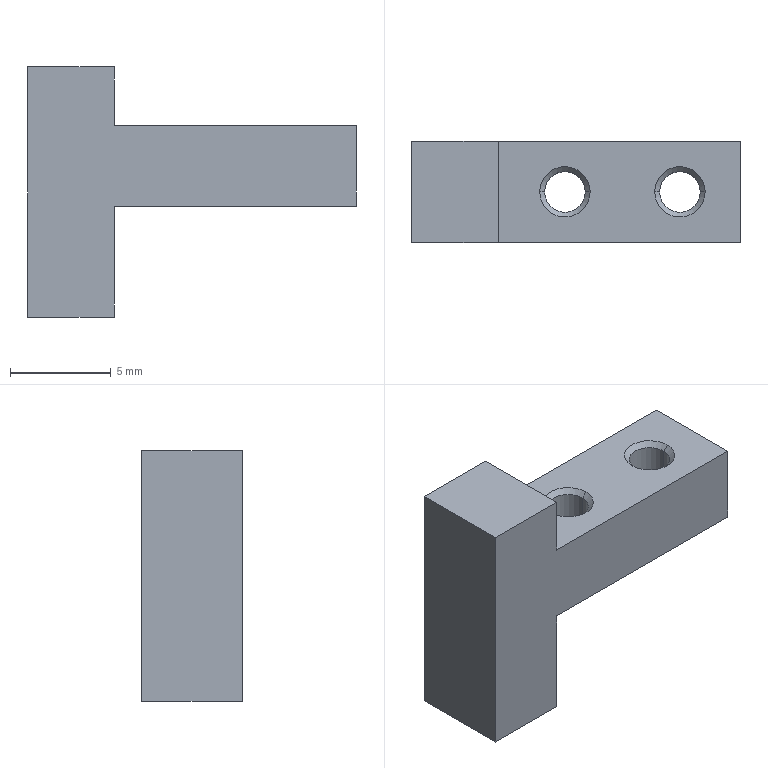Component | SolidWorks | MHZ2-10D-1_CopyCopyFinger2A_MHZ2-10D(11.2)-1 | 1 solid | 22 faces | box 16.3 x 5 x 12.4 mm | volume 480 mm3 | plane 10 | cone 8 | cylinder 4 | commonest cylinder face diameters 2.01 x4
STEP:
#1=COLOUR_RGB('',0.7922,0.8196,0.9333);
#2=FILL_AREA_STYLE_COLOUR('',#1);
#3=FILL_AREA_STYLE('',(#2));
#4=SURFACE_STYLE_FILL_AREA(#3);
#5=SURFACE_SIDE_STYLE('',(#4));
#6=SURFACE_STYLE_USAGE(.BOTH.,#5);
#7=PRESENTATION_STYLE_ASSIGNMENT((#6));
#8=CARTESIAN_POINT('',(7.83,1.719,1.739));
#9=VERTEX_POINT('',#8);
#10=CARTESIAN_POINT('',(7.751,1.719,1.739));
#11=VERTEX_POINT('',#10);
#12=CARTESIAN_POINT('',(7.79,1.719,1.739));
#13=DIRECTION('',(-0.,-0.,-1.));
#14=DIRECTION('',(1.,0.,0.));
#15=AXIS2_PLACEMENT_3D('',#12,#13,#14);
#16=CIRCLE('',#15,0.03957);
#17=EDGE_CURVE('',#9,#11,#16,.T.);
#18=ORIENTED_EDGE('',*,*,#17,.F.);
#19=CARTESIAN_POINT('',(7.839,1.719,1.73));
#20=VERTEX_POINT('',#19);
#21=CARTESIAN_POINT('',(7.839,1.719,1.73));
#22=DIRECTION('',(0.7071,-0.,-0.7071));
#23=VECTOR('',#22,39.37);
#24=LINE('',#21,#23);
#25=EDGE_CURVE('',#9,#20,#24,.T.);
#26=ORIENTED_EDGE('',*,*,#25,.T.);
#27=CARTESIAN_POINT('',(7.741,1.719,1.73));
#28=VERTEX_POINT('',#27);
#29=CARTESIAN_POINT('',(7.79,1.719,1.73));
#30=DIRECTION('',(0.,0.,1.));
#31=DIRECTION('',(-1.,0.,0.));
#32=AXIS2_PLACEMENT_3D('',#29,#30,#31);
#33=CIRCLE('',#32,0.04921);
#34=EDGE_CURVE('',#28,#20,#33,.T.);
#35=ORIENTED_EDGE('',*,*,#34,.F.);
#36=CARTESIAN_POINT('',(7.741,1.719,1.73));
#37=DIRECTION('',(-0.7071,-0.,-0.7071));
#38=VECTOR('',#37,39.37);
#39=LINE('',#36,#38);
#40=EDGE_CURVE('',#11,#28,#39,.T.);
#41=ORIENTED_EDGE('',*,*,#40,.F.);
#42=EDGE_LOOP('',(#18,#26,#35,#41));
#43=FACE_OUTER_BOUND('',#42,.T.);
#44=CARTESIAN_POINT('',(7.79,1.719,1.73));
#45=DIRECTION('',(-0.,-0.,-1.));
#46=DIRECTION('',(-1.,0.,0.));
#47=AXIS2_PLACEMENT_3D('',#44,#45,#46);
#48=CONICAL_SURFACE('',#47,0.04921,0.7854);
#49=ADVANCED_FACE('',(#43),#48,.F.);
#50=CARTESIAN_POINT('',(7.605,1.719,1.739));
#51=VERTEX_POINT('',#50);
#52=CARTESIAN_POINT('',(7.526,1.719,1.739));
#53=VERTEX_POINT('',#52);
#54=CARTESIAN_POINT('',(7.566,1.719,1.739));
#55=DIRECTION('',(-0.,-0.,-1.));
#56=DIRECTION('',(1.,0.,0.));
#57=AXIS2_PLACEMENT_3D('',#54,#55,#56);
#58=CIRCLE('',#57,0.03957);
#59=EDGE_CURVE('',#51,#53,#58,.T.);
#60=ORIENTED_EDGE('',*,*,#59,.F.);
#61=CARTESIAN_POINT('',(7.615,1.719,1.73));
#62=VERTEX_POINT('',#61);
#63=CARTESIAN_POINT('',(7.615,1.719,1.73));
#64=DIRECTION('',(0.7071,-0.,-0.7071));
#65=VECTOR('',#64,39.37);
#66=LINE('',#63,#65);
#67=EDGE_CURVE('',#51,#62,#66,.T.);
#68=ORIENTED_EDGE('',*,*,#67,.T.);
#69=CARTESIAN_POINT('',(7.517,1.719,1.73));
#70=VERTEX_POINT('',#69);
#71=CARTESIAN_POINT('',(7.566,1.719,1.73));
#72=DIRECTION('',(0.,0.,1.));
#73=DIRECTION('',(-1.,0.,0.));
#74=AXIS2_PLACEMENT_3D('',#71,#72,#73);
#75=CIRCLE('',#74,0.04921);
#76=EDGE_CURVE('',#70,#62,#75,.T.);
#77=ORIENTED_EDGE('',*,*,#76,.F.);
#78=CARTESIAN_POINT('',(7.517,1.719,1.73));
#79=DIRECTION('',(-0.7071,-0.,-0.7071));
#80=VECTOR('',#79,39.37);
#81=LINE('',#78,#80);
#82=EDGE_CURVE('',#53,#70,#81,.T.);
#83=ORIENTED_EDGE('',*,*,#82,.F.);
#84=EDGE_LOOP('',(#60,#68,#77,#83));
#85=FACE_OUTER_BOUND('',#84,.T.);
#86=CARTESIAN_POINT('',(7.566,1.719,1.73));
#87=DIRECTION('',(-0.,-0.,-1.));
#88=DIRECTION('',(-1.,0.,0.));
#89=AXIS2_PLACEMENT_3D('',#86,#87,#88);
#90=CONICAL_SURFACE('',#89,0.04921,0.7854);
#91=ADVANCED_FACE('',(#85),#90,.F.);
#92=CARTESIAN_POINT('',(7.751,1.719,1.877));
#93=VERTEX_POINT('',#92);
#94=CARTESIAN_POINT('',(7.83,1.719,1.877));
#95=VERTEX_POINT('',#94);
#96=CARTESIAN_POINT('',(7.79,1.719,1.877));
#97=DIRECTION('',(0.,0.,1.));
#98=DIRECTION('',(1.,0.,0.));
#99=AXIS2_PLACEMENT_3D('',#96,#97,#98);
#100=CIRCLE('',#99,0.03957);
#101=EDGE_CURVE('',#93,#95,#100,.T.);
#102=ORIENTED_EDGE('',*,*,#101,.F.);
#103=CARTESIAN_POINT('',(7.741,1.719,1.887));
#104=VERTEX_POINT('',#103);
#105=CARTESIAN_POINT('',(7.741,1.719,1.887));
#106=DIRECTION('',(-0.7071,0.,0.7071));
#107=VECTOR('',#106,39.37);
#108=LINE('',#105,#107);
#109=EDGE_CURVE('',#93,#104,#108,.T.);
#110=ORIENTED_EDGE('',*,*,#109,.T.);
#111=CARTESIAN_POINT('',(7.839,1.719,1.887));
#112=VERTEX_POINT('',#111);
#113=CARTESIAN_POINT('',(7.79,1.719,1.887));
#114=DIRECTION('',(-0.,-0.,-1.));
#115=DIRECTION('',(1.,0.,0.));
#116=AXIS2_PLACEMENT_3D('',#113,#114,#115);
#117=CIRCLE('',#116,0.04921);
#118=EDGE_CURVE('',#112,#104,#117,.T.);
#119=ORIENTED_EDGE('',*,*,#118,.F.);
#120=CARTESIAN_POINT('',(7.839,1.719,1.887));
#121=DIRECTION('',(0.7071,0.,0.7071));
#122=VECTOR('',#121,39.37);
#123=LINE('',#120,#122);
#124=EDGE_CURVE('',#95,#112,#123,.T.);
#125=ORIENTED_EDGE('',*,*,#124,.F.);
#126=EDGE_LOOP('',(#102,#110,#119,#125));
#127=FACE_OUTER_BOUND('',#126,.T.);
#128=CARTESIAN_POINT('',(7.79,1.719,1.887));
#129=DIRECTION('',(0.,0.,1.));
#130=DIRECTION('',(1.,0.,0.));
#131=AXIS2_PLACEMENT_3D('',#128,#129,#130);
#132=CONICAL_SURFACE('',#131,0.04921,0.7854);
#133=ADVANCED_FACE('',(#127),#132,.F.);
#134=CARTESIAN_POINT('',(7.526,1.719,1.877));
#135=VERTEX_POINT('',#134);
#136=CARTESIAN_POINT('',(7.605,1.719,1.877));
#137=VERTEX_POINT('',#136);
#138=CARTESIAN_POINT('',(7.566,1.719,1.877));
#139=DIRECTION('',(0.,0.,1.));
#140=DIRECTION('',(1.,0.,0.));
#141=AXIS2_PLACEMENT_3D('',#138,#139,#140);
#142=CIRCLE('',#141,0.03957);
#143=EDGE_CURVE('',#135,#137,#142,.T.);
#144=ORIENTED_EDGE('',*,*,#143,.F.);
#145=CARTESIAN_POINT('',(7.517,1.719,1.887));
#146=VERTEX_POINT('',#145);
#147=CARTESIAN_POINT('',(7.517,1.719,1.887));
#148=DIRECTION('',(-0.7071,0.,0.7071));
#149=VECTOR('',#148,39.37);
#150=LINE('',#147,#149);
#151=EDGE_CURVE('',#135,#146,#150,.T.);
#152=ORIENTED_EDGE('',*,*,#151,.T.);
#153=CARTESIAN_POINT('',(7.615,1.719,1.887));
#154=VERTEX_POINT('',#153);
#155=CARTESIAN_POINT('',(7.566,1.719,1.887));
#156=DIRECTION('',(-0.,-0.,-1.));
#157=DIRECTION('',(1.,0.,0.));
#158=AXIS2_PLACEMENT_3D('',#155,#156,#157);
#159=CIRCLE('',#158,0.04921);
#160=EDGE_CURVE('',#154,#146,#159,.T.);
#161=ORIENTED_EDGE('',*,*,#160,.F.);
#162=CARTESIAN_POINT('',(7.615,1.719,1.887));
#163=DIRECTION('',(0.7071,0.,0.7071));
#164=VECTOR('',#163,39.37);
#165=LINE('',#162,#164);
#166=EDGE_CURVE('',#137,#154,#165,.T.);
#167=ORIENTED_EDGE('',*,*,#166,.F.);
#168=EDGE_LOOP('',(#144,#152,#161,#167));
#169=FACE_OUTER_BOUND('',#168,.T.);
#170=CARTESIAN_POINT('',(7.566,1.719,1.887));
#171=DIRECTION('',(0.,0.,1.));
#172=DIRECTION('',(1.,0.,0.));
#173=AXIS2_PLACEMENT_3D('',#170,#171,#172);
#174=CONICAL_SURFACE('',#173,0.04921,0.7854);
#175=ADVANCED_FACE('',(#169),#174,.F.);
#176=ORIENTED_EDGE('',*,*,#101,.T.);
#177=CARTESIAN_POINT('',(7.83,1.719,1.808));
#178=DIRECTION('',(-0.,-0.,-1.));
#179=VECTOR('',#178,39.37);
#180=LINE('',#177,#179);
#181=EDGE_CURVE('',#95,#9,#180,.T.);
#182=ORIENTED_EDGE('',*,*,#181,.T.);
#183=ORIENTED_EDGE('',*,*,#17,.T.);
#184=CARTESIAN_POINT('',(7.751,1.719,1.808));
#185=DIRECTION('',(-0.,-0.,-1.));
#186=VECTOR('',#185,39.37);
#187=LINE('',#184,#186);
#188=EDGE_CURVE('',#93,#11,#187,.T.);
#189=ORIENTED_EDGE('',*,*,#188,.F.);
#190=EDGE_LOOP('',(#176,#182,#183,#189));
#191=FACE_OUTER_BOUND('',#190,.T.);
#192=CARTESIAN_POINT('',(7.79,1.719,1.808));
#193=DIRECTION('',(-0.,-0.,-1.));
#194=DIRECTION('',(-1.,0.,0.));
#195=AXIS2_PLACEMENT_3D('',#192,#193,#194);
#196=CYLINDRICAL_SURFACE('',#195,0.03957);
#197=ADVANCED_FACE('',(#191),#196,.F.);
#198=ORIENTED_EDGE('',*,*,#143,.T.);
#199=CARTESIAN_POINT('',(7.605,1.719,1.808));
#200=DIRECTION('',(-0.,-0.,-1.));
#201=VECTOR('',#200,39.37);
#202=LINE('',#199,#201);
#203=EDGE_CURVE('',#137,#51,#202,.T.);
#204=ORIENTED_EDGE('',*,*,#203,.T.);
#205=ORIENTED_EDGE('',*,*,#59,.T.);
#206=CARTESIAN_POINT('',(7.526,1.719,1.808));
#207=DIRECTION('',(-0.,-0.,-1.));
#208=VECTOR('',#207,39.37);
#209=LINE('',#206,#208);
#210=EDGE_CURVE('',#135,#53,#209,.T.);
#211=ORIENTED_EDGE('',*,*,#210,.F.);
#212=EDGE_LOOP('',(#198,#204,#205,#211));
#213=FACE_OUTER_BOUND('',#212,.T.);
#214=CARTESIAN_POINT('',(7.566,1.719,1.808));
#215=DIRECTION('',(-0.,-0.,-1.));
#216=DIRECTION('',(-1.,0.,0.));
#217=AXIS2_PLACEMENT_3D('',#214,#215,#216);
#218=CYLINDRICAL_SURFACE('',#217,0.03957);
#219=ADVANCED_FACE('',(#213),#218,.F.);
#220=CARTESIAN_POINT('',(7.267,1.818,1.513));
#221=VERTEX_POINT('',#220);
#222=CARTESIAN_POINT('',(7.267,1.818,2.001));
#223=VERTEX_POINT('',#222);
#224=CARTESIAN_POINT('',(7.267,1.818,1.509));
#225=DIRECTION('',(0.,0.,1.));
#226=VECTOR('',#225,39.37);
#227=LINE('',#224,#226);
#228=EDGE_CURVE('',#221,#223,#227,.T.);
#229=ORIENTED_EDGE('',*,*,#228,.T.);
#230=CARTESIAN_POINT('',(7.436,1.818,2.001));
#231=VERTEX_POINT('',#230);
#232=CARTESIAN_POINT('',(7.389,1.818,2.001));
#233=DIRECTION('',(1.,0.,-0.));
#234=VECTOR('',#233,39.37);
#235=LINE('',#232,#234);
#236=EDGE_CURVE('',#223,#231,#235,.T.);
#237=ORIENTED_EDGE('',*,*,#236,.T.);
#238=CARTESIAN_POINT('',(7.436,1.818,1.887));
#239=VERTEX_POINT('',#238);
#240=CARTESIAN_POINT('',(7.436,1.818,1.509));
#241=DIRECTION('',(-0.,-0.,-1.));
#242=VECTOR('',#241,39.37);
#243=LINE('',#240,#242);
#244=EDGE_CURVE('',#231,#239,#243,.T.);
#245=ORIENTED_EDGE('',*,*,#244,.T.);
#246=CARTESIAN_POINT('',(7.908,1.818,1.887));
#247=VERTEX_POINT('',#246);
#248=CARTESIAN_POINT('',(7.389,1.818,1.887));
#249=DIRECTION('',(1.,0.,-0.));
#250=VECTOR('',#249,39.37);
#251=LINE('',#248,#250);
#252=EDGE_CURVE('',#239,#247,#251,.T.);
#253=ORIENTED_EDGE('',*,*,#252,.T.);
#254=CARTESIAN_POINT('',(7.908,1.818,1.73));
#255=VERTEX_POINT('',#254);
#256=CARTESIAN_POINT('',(7.908,1.818,1.509));
#257=DIRECTION('',(-0.,-0.,-1.));
#258=VECTOR('',#257,39.37);
#259=LINE('',#256,#258);
#260=EDGE_CURVE('',#247,#255,#259,.T.);
#261=ORIENTED_EDGE('',*,*,#260,.T.);
#262=CARTESIAN_POINT('',(7.436,1.818,1.73));
#263=VERTEX_POINT('',#262);
#264=CARTESIAN_POINT('',(7.389,1.818,1.73));
#265=DIRECTION('',(-1.,-0.,0.));
#266=VECTOR('',#265,39.37);
#267=LINE('',#264,#266);
#268=EDGE_CURVE('',#255,#263,#267,.T.);
#269=ORIENTED_EDGE('',*,*,#268,.T.);
#270=CARTESIAN_POINT('',(7.436,1.818,1.513));
#271=VERTEX_POINT('',#270);
#272=CARTESIAN_POINT('',(7.436,1.818,1.509));
#273=DIRECTION('',(-0.,-0.,-1.));
#274=VECTOR('',#273,39.37);
#275=LINE('',#272,#274);
#276=EDGE_CURVE('',#263,#271,#275,.T.);
#277=ORIENTED_EDGE('',*,*,#276,.T.);
#278=CARTESIAN_POINT('',(7.389,1.818,1.513));
#279=DIRECTION('',(-1.,-0.,0.));
#280=VECTOR('',#279,39.37);
#281=LINE('',#278,#280);
#282=EDGE_CURVE('',#271,#221,#281,.T.);
#283=ORIENTED_EDGE('',*,*,#282,.T.);
#284=EDGE_LOOP('',(#229,#237,#245,#253,#261,#269,#277,#283));
#285=FACE_OUTER_BOUND('',#284,.T.);
#286=CARTESIAN_POINT('',(7.389,1.818,1.509));
#287=DIRECTION('',(-0.,1.,-0.));
#288=DIRECTION('',(1.,0.,-0.));
#289=AXIS2_PLACEMENT_3D('',#286,#287,#288);
#290=PLANE('',#289);
#291=ADVANCED_FACE('',(#285),#290,.T.);
#292=ORIENTED_EDGE('',*,*,#236,.F.);
#293=CARTESIAN_POINT('',(7.267,1.621,2.001));
#294=VERTEX_POINT('',#293);
#295=CARTESIAN_POINT('',(7.267,1.818,2.001));
#296=DIRECTION('',(0.,-1.,0.));
#297=VECTOR('',#296,39.37);
#298=LINE('',#295,#297);
#299=EDGE_CURVE('',#223,#294,#298,.T.);
#300=ORIENTED_EDGE('',*,*,#299,.T.);
#301=CARTESIAN_POINT('',(7.436,1.621,2.001));
#302=VERTEX_POINT('',#301);
#303=CARTESIAN_POINT('',(7.267,1.621,2.001));
#304=DIRECTION('',(1.,0.,-0.));
#305=VECTOR('',#304,39.37);
#306=LINE('',#303,#305);
#307=EDGE_CURVE('',#294,#302,#306,.T.);
#308=ORIENTED_EDGE('',*,*,#307,.T.);
#309=CARTESIAN_POINT('',(7.436,1.818,2.001));
#310=DIRECTION('',(-0.,1.,-0.));
#311=VECTOR('',#310,39.37);
#312=LINE('',#309,#311);
#313=EDGE_CURVE('',#302,#231,#312,.T.);
#314=ORIENTED_EDGE('',*,*,#313,.T.);
#315=EDGE_LOOP('',(#292,#300,#308,#314));
#316=FACE_OUTER_BOUND('',#315,.T.);
#317=CARTESIAN_POINT('',(7.267,1.818,2.001));
#318=DIRECTION('',(0.,0.,1.));
#319=DIRECTION('',(1.,0.,-0.));
#320=AXIS2_PLACEMENT_3D('',#317,#318,#319);
#321=PLANE('',#320);
#322=ADVANCED_FACE('',(#316),#321,.T.);
#323=ORIENTED_EDGE('',*,*,#228,.F.);
#324=CARTESIAN_POINT('',(7.267,1.621,1.513));
#325=VERTEX_POINT('',#324);
#326=CARTESIAN_POINT('',(7.267,1.818,1.513));
#327=DIRECTION('',(0.,-1.,0.));
#328=VECTOR('',#327,39.37);
#329=LINE('',#326,#328);
#330=EDGE_CURVE('',#221,#325,#329,.T.);
#331=ORIENTED_EDGE('',*,*,#330,.T.);
#332=CARTESIAN_POINT('',(7.267,1.621,1.513));
#333=DIRECTION('',(-0.,0.,1.));
#334=VECTOR('',#333,39.37);
#335=LINE('',#332,#334);
#336=EDGE_CURVE('',#325,#294,#335,.T.);
#337=ORIENTED_EDGE('',*,*,#336,.T.);
#338=ORIENTED_EDGE('',*,*,#299,.F.);
#339=EDGE_LOOP('',(#323,#331,#337,#338));
#340=FACE_OUTER_BOUND('',#339,.T.);
#341=CARTESIAN_POINT('',(7.267,1.818,1.513));
#342=DIRECTION('',(-1.,-0.,-0.));
#343=DIRECTION('',(-0.,0.,1.));
#344=AXIS2_PLACEMENT_3D('',#341,#342,#343);
#345=PLANE('',#344);
#346=ADVANCED_FACE('',(#340),#345,.T.);
#347=ORIENTED_EDGE('',*,*,#282,.F.);
#348=CARTESIAN_POINT('',(7.436,1.621,1.513));
#349=VERTEX_POINT('',#348);
#350=CARTESIAN_POINT('',(7.436,1.818,1.513));
#351=DIRECTION('',(0.,-1.,0.));
#352=VECTOR('',#351,39.37);
#353=LINE('',#350,#352);
#354=EDGE_CURVE('',#271,#349,#353,.T.);
#355=ORIENTED_EDGE('',*,*,#354,.T.);
#356=CARTESIAN_POINT('',(7.436,1.621,1.513));
#357=DIRECTION('',(-1.,-0.,0.));
#358=VECTOR('',#357,39.37);
#359=LINE('',#356,#358);
#360=EDGE_CURVE('',#349,#325,#359,.T.);
#361=ORIENTED_EDGE('',*,*,#360,.T.);
#362=ORIENTED_EDGE('',*,*,#330,.F.);
#363=EDGE_LOOP('',(#347,#355,#361,#362));
#364=FACE_OUTER_BOUND('',#363,.T.);
#365=CARTESIAN_POINT('',(7.436,1.818,1.513));
#366=DIRECTION('',(-0.,-0.,-1.));
#367=DIRECTION('',(-1.,-0.,0.));
#368=AXIS2_PLACEMENT_3D('',#365,#366,#367);
#369=PLANE('',#368);
#370=ADVANCED_FACE('',(#364),#369,.T.);
#371=ORIENTED_EDGE('',*,*,#276,.F.);
#372=CARTESIAN_POINT('',(7.436,1.621,1.73));
#373=VERTEX_POINT('',#372);
#374=CARTESIAN_POINT('',(7.436,1.818,1.73));
#375=DIRECTION('',(0.,-1.,0.));
#376=VECTOR('',#375,39.37);
#377=LINE('',#374,#376);
#378=EDGE_CURVE('',#263,#373,#377,.T.);
#379=ORIENTED_EDGE('',*,*,#378,.T.);
#380=CARTESIAN_POINT('',(7.436,1.621,1.73));
#381=DIRECTION('',(-0.,-0.,-1.));
#382=VECTOR('',#381,39.37);
#383=LINE('',#380,#382);
#384=EDGE_CURVE('',#373,#349,#383,.T.);
#385=ORIENTED_EDGE('',*,*,#384,.T.);
#386=ORIENTED_EDGE('',*,*,#354,.F.);
#387=EDGE_LOOP('',(#371,#379,#385,#386));
#388=FACE_OUTER_BOUND('',#387,.T.);
#389=CARTESIAN_POINT('',(7.436,1.818,1.73));
#390=DIRECTION('',(1.,0.,-0.));
#391=DIRECTION('',(0.,-1.,0.));
#392=AXIS2_PLACEMENT_3D('',#389,#390,#391);
#393=PLANE('',#392);
#394=ADVANCED_FACE('',(#388),#393,.T.);
#395=ORIENTED_EDGE('',*,*,#268,.F.);
#396=CARTESIAN_POINT('',(7.908,1.621,1.73));
#397=VERTEX_POINT('',#396);
#398=CARTESIAN_POINT('',(7.908,1.818,1.73));
#399=DIRECTION('',(0.,-1.,0.));
#400=VECTOR('',#399,39.37);
#401=LINE('',#398,#400);
#402=EDGE_CURVE('',#255,#397,#401,.T.);
#403=ORIENTED_EDGE('',*,*,#402,.T.);
#404=CARTESIAN_POINT('',(7.908,1.621,1.73));
#405=DIRECTION('',(-1.,-0.,0.));
#406=VECTOR('',#405,39.37);
#407=LINE('',#404,#406);
#408=EDGE_CURVE('',#397,#373,#407,.T.);
#409=ORIENTED_EDGE('',*,*,#408,.T.);
#410=ORIENTED_EDGE('',*,*,#378,.F.);
#411=EDGE_LOOP('',(#395,#403,#409,#410));
#412=FACE_OUTER_BOUND('',#411,.T.);
#413=ORIENTED_EDGE('',*,*,#34,.T.);
#414=CARTESIAN_POINT('',(7.79,1.719,1.73));
#415=DIRECTION('',(0.,0.,1.));
#416=DIRECTION('',(-1.,0.,0.));
#417=AXIS2_PLACEMENT_3D('',#414,#415,#416);
#418=CIRCLE('',#417,0.04921);
#419=EDGE_CURVE('',#20,#28,#418,.T.);
#420=ORIENTED_EDGE('',*,*,#419,.T.);
#421=EDGE_LOOP('',(#413,#420));
#422=FACE_BOUND('',#421,.T.);
#423=ORIENTED_EDGE('',*,*,#76,.T.);
#424=CARTESIAN_POINT('',(7.566,1.719,1.73));
#425=DIRECTION('',(0.,0.,1.));
#426=DIRECTION('',(-1.,0.,0.));
#427=AXIS2_PLACEMENT_3D('',#424,#425,#426);
#428=CIRCLE('',#427,0.04921);
#429=EDGE_CURVE('',#62,#70,#428,.T.);
#430=ORIENTED_EDGE('',*,*,#429,.T.);
#431=EDGE_LOOP('',(#423,#430));
#432=FACE_BOUND('',#431,.T.);
#433=CARTESIAN_POINT('',(7.908,1.818,1.73));
#434=DIRECTION('',(-0.,-0.,-1.));
#435=DIRECTION('',(-1.,-0.,0.));
#436=AXIS2_PLACEMENT_3D('',#433,#434,#435);
#437=PLANE('',#436);
#438=ADVANCED_FACE('',(#412,#422,#432),#437,.T.);
#439=ORIENTED_EDGE('',*,*,#260,.F.);
#440=CARTESIAN_POINT('',(7.908,1.621,1.887));
#441=VERTEX_POINT('',#440);
#442=CARTESIAN_POINT('',(7.908,1.818,1.887));
#443=DIRECTION('',(0.,-1.,0.));
#444=VECTOR('',#443,39.37);
#445=LINE('',#442,#444);
#446=EDGE_CURVE('',#247,#441,#445,.T.);
#447=ORIENTED_EDGE('',*,*,#446,.T.);
#448=CARTESIAN_POINT('',(7.908,1.621,1.887));
#449=DIRECTION('',(-0.,-0.,-1.));
#450=VECTOR('',#449,39.37);
#451=LINE('',#448,#450);
#452=EDGE_CURVE('',#441,#397,#451,.T.);
#453=ORIENTED_EDGE('',*,*,#452,.T.);
#454=ORIENTED_EDGE('',*,*,#402,.F.);
#455=EDGE_LOOP('',(#439,#447,#453,#454));
#456=FACE_OUTER_BOUND('',#455,.T.);
#457=CARTESIAN_POINT('',(7.908,1.818,1.887));
#458=DIRECTION('',(1.,0.,-0.));
#459=DIRECTION('',(-0.,-0.,-1.));
#460=AXIS2_PLACEMENT_3D('',#457,#458,#459);
#461=PLANE('',#460);
#462=ADVANCED_FACE('',(#456),#461,.T.);
#463=ORIENTED_EDGE('',*,*,#252,.F.);
#464=CARTESIAN_POINT('',(7.436,1.621,1.887));
#465=VERTEX_POINT('',#464);
#466=CARTESIAN_POINT('',(7.436,1.818,1.887));
#467=DIRECTION('',(0.,-1.,0.));
#468=VECTOR('',#467,39.37);
#469=LINE('',#466,#468);
#470=EDGE_CURVE('',#239,#465,#469,.T.);
#471=ORIENTED_EDGE('',*,*,#470,.T.);
#472=CARTESIAN_POINT('',(7.436,1.621,1.887));
#473=DIRECTION('',(1.,0.,-0.));
#474=VECTOR('',#473,39.37);
#475=LINE('',#472,#474);
#476=EDGE_CURVE('',#465,#441,#475,.T.);
#477=ORIENTED_EDGE('',*,*,#476,.T.);
#478=ORIENTED_EDGE('',*,*,#446,.F.);
#479=EDGE_LOOP('',(#463,#471,#477,#478));
#480=FACE_OUTER_BOUND('',#479,.T.);
#481=ORIENTED_EDGE('',*,*,#118,.T.);
#482=CARTESIAN_POINT('',(7.79,1.719,1.887));
#483=DIRECTION('',(-0.,-0.,-1.));
#484=DIRECTION('',(1.,0.,0.));
#485=AXIS2_PLACEMENT_3D('',#482,#483,#484);
#486=CIRCLE('',#485,0.04921);
#487=EDGE_CURVE('',#104,#112,#486,.T.);
#488=ORIENTED_EDGE('',*,*,#487,.T.);
#489=EDGE_LOOP('',(#481,#488));
#490=FACE_BOUND('',#489,.T.);
#491=ORIENTED_EDGE('',*,*,#160,.T.);
#492=CARTESIAN_POINT('',(7.566,1.719,1.887));
#493=DIRECTION('',(-0.,-0.,-1.));
#494=DIRECTION('',(1.,0.,0.));
#495=AXIS2_PLACEMENT_3D('',#492,#493,#494);
#496=CIRCLE('',#495,0.04921);
#497=EDGE_CURVE('',#146,#154,#496,.T.);
#498=ORIENTED_EDGE('',*,*,#497,.T.);
#499=EDGE_LOOP('',(#491,#498));
#500=FACE_BOUND('',#499,.T.);
#501=CARTESIAN_POINT('',(7.436,1.818,1.887));
#502=DIRECTION('',(0.,0.,1.));
#503=DIRECTION('',(1.,0.,-0.));
#504=AXIS2_PLACEMENT_3D('',#501,#502,#503);
#505=PLANE('',#504);
#506=ADVANCED_FACE('',(#480,#490,#500),#505,.T.);
#507=ORIENTED_EDGE('',*,*,#244,.F.);
#508=ORIENTED_EDGE('',*,*,#313,.F.);
#509=CARTESIAN_POINT('',(7.436,1.621,2.001));
#510=DIRECTION('',(-0.,-0.,-1.));
#511=VECTOR('',#510,39.37);
#512=LINE('',#509,#511);
#513=EDGE_CURVE('',#302,#465,#512,.T.);
#514=ORIENTED_EDGE('',*,*,#513,.T.);
#515=ORIENTED_EDGE('',*,*,#470,.F.);
#516=EDGE_LOOP('',(#507,#508,#514,#515));
#517=FACE_OUTER_BOUND('',#516,.T.);
#518=CARTESIAN_POINT('',(7.436,1.818,2.001));
#519=DIRECTION('',(1.,0.,-0.));
#520=DIRECTION('',(0.,-1.,0.));
#521=AXIS2_PLACEMENT_3D('',#518,#519,#520);
#522=PLANE('',#521);
#523=ADVANCED_FACE('',(#517),#522,.T.);
#524=ORIENTED_EDGE('',*,*,#513,.F.);
#525=ORIENTED_EDGE('',*,*,#307,.F.);
#526=ORIENTED_EDGE('',*,*,#336,.F.);
#527=ORIENTED_EDGE('',*,*,#360,.F.);
#528=ORIENTED_EDGE('',*,*,#384,.F.);
#529=ORIENTED_EDGE('',*,*,#408,.F.);
#530=ORIENTED_EDGE('',*,*,#452,.F.);
#531=ORIENTED_EDGE('',*,*,#476,.F.);
#532=EDGE_LOOP('',(#524,#525,#526,#527,#528,#529,#530,#531));
#533=FACE_OUTER_BOUND('',#532,.T.);
#534=CARTESIAN_POINT('',(7.389,1.621,1.509));
#535=DIRECTION('',(-0.,1.,-0.));
#536=DIRECTION('',(1.,0.,-0.));
#537=AXIS2_PLACEMENT_3D('',#534,#535,#536);
#538=PLANE('',#537);
#539=ADVANCED_FACE('',(#533),#538,.F.);
#540=ORIENTED_EDGE('',*,*,#25,.F.);
#541=CARTESIAN_POINT('',(7.79,1.719,1.739));
#542=DIRECTION('',(-0.,-0.,-1.));
#543=DIRECTION('',(1.,0.,0.));
#544=AXIS2_PLACEMENT_3D('',#541,#542,#543);
#545=CIRCLE('',#544,0.03957);
#546=EDGE_CURVE('',#11,#9,#545,.T.);
#547=ORIENTED_EDGE('',*,*,#546,.F.);
#548=ORIENTED_EDGE('',*,*,#40,.T.);
#549=ORIENTED_EDGE('',*,*,#419,.F.);
#550=EDGE_LOOP('',(#540,#547,#548,#549));
#551=FACE_OUTER_BOUND('',#550,.T.);
#552=CARTESIAN_POINT('',(7.79,1.719,1.73));
#553=DIRECTION('',(-0.,-0.,-1.));
#554=DIRECTION('',(-1.,0.,0.));
#555=AXIS2_PLACEMENT_3D('',#552,#553,#554);
#556=CONICAL_SURFACE('',#555,0.04921,0.7854);
#557=ADVANCED_FACE('',(#551),#556,.F.);
#558=ORIENTED_EDGE('',*,*,#67,.F.);
#559=CARTESIAN_POINT('',(7.566,1.719,1.739));
#560=DIRECTION('',(-0.,-0.,-1.));
#561=DIRECTION('',(1.,0.,0.));
#562=AXIS2_PLACEMENT_3D('',#559,#560,#561);
#563=CIRCLE('',#562,0.03957);
#564=EDGE_CURVE('',#53,#51,#563,.T.);
#565=ORIENTED_EDGE('',*,*,#564,.F.);
#566=ORIENTED_EDGE('',*,*,#82,.T.);
#567=ORIENTED_EDGE('',*,*,#429,.F.);
#568=EDGE_LOOP('',(#558,#565,#566,#567));
#569=FACE_OUTER_BOUND('',#568,.T.);
#570=CARTESIAN_POINT('',(7.566,1.719,1.73));
#571=DIRECTION('',(-0.,-0.,-1.));
#572=DIRECTION('',(-1.,0.,0.));
#573=AXIS2_PLACEMENT_3D('',#570,#571,#572);
#574=CONICAL_SURFACE('',#573,0.04921,0.7854);
#575=ADVANCED_FACE('',(#569),#574,.F.);
#576=ORIENTED_EDGE('',*,*,#109,.F.);
#577=CARTESIAN_POINT('',(7.79,1.719,1.877));
#578=DIRECTION('',(0.,0.,1.));
#579=DIRECTION('',(1.,0.,0.));
#580=AXIS2_PLACEMENT_3D('',#577,#578,#579);
#581=CIRCLE('',#580,0.03957);
#582=EDGE_CURVE('',#95,#93,#581,.T.);
#583=ORIENTED_EDGE('',*,*,#582,.F.);
#584=ORIENTED_EDGE('',*,*,#124,.T.);
#585=ORIENTED_EDGE('',*,*,#487,.F.);
#586=EDGE_LOOP('',(#576,#583,#584,#585));
#587=FACE_OUTER_BOUND('',#586,.T.);
#588=CARTESIAN_POINT('',(7.79,1.719,1.887));
#589=DIRECTION('',(0.,0.,1.));
#590=DIRECTION('',(1.,0.,0.));
#591=AXIS2_PLACEMENT_3D('',#588,#589,#590);
#592=CONICAL_SURFACE('',#591,0.04921,0.7854);
#593=ADVANCED_FACE('',(#587),#592,.F.);
#594=ORIENTED_EDGE('',*,*,#151,.F.);
#595=CARTESIAN_POINT('',(7.566,1.719,1.877));
#596=DIRECTION('',(0.,0.,1.));
#597=DIRECTION('',(1.,0.,0.));
#598=AXIS2_PLACEMENT_3D('',#595,#596,#597);
#599=CIRCLE('',#598,0.03957);
#600=EDGE_CURVE('',#137,#135,#599,.T.);
#601=ORIENTED_EDGE('',*,*,#600,.F.);
#602=ORIENTED_EDGE('',*,*,#166,.T.);
#603=ORIENTED_EDGE('',*,*,#497,.F.);
#604=EDGE_LOOP('',(#594,#601,#602,#603));
#605=FACE_OUTER_BOUND('',#604,.T.);
#606=CARTESIAN_POINT('',(7.566,1.719,1.887));
#607=DIRECTION('',(0.,0.,1.));
#608=DIRECTION('',(1.,0.,0.));
#609=AXIS2_PLACEMENT_3D('',#606,#607,#608);
#610=CONICAL_SURFACE('',#609,0.04921,0.7854);
#611=ADVANCED_FACE('',(#605),#610,.F.);
#612=ORIENTED_EDGE('',*,*,#181,.F.);
#613=ORIENTED_EDGE('',*,*,#582,.T.);
#614=ORIENTED_EDGE('',*,*,#188,.T.);
#615=ORIENTED_EDGE('',*,*,#546,.T.);
#616=EDGE_LOOP('',(#612,#613,#614,#615));
#617=FACE_OUTER_BOUND('',#616,.T.);
#618=CARTESIAN_POINT('',(7.79,1.719,1.808));
#619=DIRECTION('',(-0.,-0.,-1.));
#620=DIRECTION('',(-1.,0.,0.));
#621=AXIS2_PLACEMENT_3D('',#618,#619,#620);
#622=CYLINDRICAL_SURFACE('',#621,0.03957);
#623=ADVANCED_FACE('',(#617),#622,.F.);
#624=ORIENTED_EDGE('',*,*,#203,.F.);
#625=ORIENTED_EDGE('',*,*,#600,.T.);
#626=ORIENTED_EDGE('',*,*,#210,.T.);
#627=ORIENTED_EDGE('',*,*,#564,.T.);
#628=EDGE_LOOP('',(#624,#625,#626,#627));
#629=FACE_OUTER_BOUND('',#628,.T.);
#630=CARTESIAN_POINT('',(7.566,1.719,1.808));
#631=DIRECTION('',(-0.,-0.,-1.));
#632=DIRECTION('',(-1.,0.,0.));
#633=AXIS2_PLACEMENT_3D('',#630,#631,#632);
#634=CYLINDRICAL_SURFACE('',#633,0.03957);
#635=ADVANCED_FACE('',(#629),#634,.F.);
#636=CLOSED_SHELL('',(#49,#91,#133,#175,#197,#219,#291,#322,#346,#370,#394,#438,#462,#506,#523,#539,#557,#575,#593,#611,#623,#635));
#637=MANIFOLD_SOLID_BREP('',#636);
#638=STYLED_ITEM('',(#7),#637);
#639=(LENGTH_UNIT()NAMED_UNIT(*)SI_UNIT($,.METRE.));
#640=LENGTH_MEASURE_WITH_UNIT(LENGTH_MEASURE(0.0254),#639);
#641=DIMENSIONAL_EXPONENTS(1.,0.,0.,0.,0.,0.,0.);
#642=(CONVERSION_BASED_UNIT('',#640)LENGTH_UNIT()NAMED_UNIT(#641));
#643=UNCERTAINTY_MEASURE_WITH_UNIT(LENGTH_MEASURE(0.00001),#642,'','');
#644=(NAMED_UNIT(*)PLANE_ANGLE_UNIT()SI_UNIT($,.RADIAN.));
#645=(NAMED_UNIT(*)SI_UNIT($,.STERADIAN.)SOLID_ANGLE_UNIT());
#646=(GEOMETRIC_REPRESENTATION_CONTEXT(3)GLOBAL_UNCERTAINTY_ASSIGNED_CONTEXT((#643))GLOBAL_UNIT_ASSIGNED_CONTEXT((#642,#644,#645))REPRESENTATION_CONTEXT('',''));
#647=MECHANICAL_DESIGN_GEOMETRIC_PRESENTATION_REPRESENTATION('',(#638),#646);
#648=CARTESIAN_POINT('',(0.,0.,0.));
#649=DIRECTION('',(0.,0.,1.));
#650=DIRECTION('',(1.,0.,0.));
#651=AXIS2_PLACEMENT_3D('',#648,#649,#650);
#652=(LENGTH_UNIT()NAMED_UNIT(*)SI_UNIT($,.METRE.));
#653=LENGTH_MEASURE_WITH_UNIT(LENGTH_MEASURE(0.0254),#652);
#654=DIMENSIONAL_EXPONENTS(1.,0.,0.,0.,0.,0.,0.);
#655=(CONVERSION_BASED_UNIT('',#653)LENGTH_UNIT()NAMED_UNIT(#654));
#656=UNCERTAINTY_MEASURE_WITH_UNIT(LENGTH_MEASURE(0.00001),#655,'','');
#657=(NAMED_UNIT(*)PLANE_ANGLE_UNIT()SI_UNIT($,.RADIAN.));
#658=(NAMED_UNIT(*)SI_UNIT($,.STERADIAN.)SOLID_ANGLE_UNIT());
#659=(GEOMETRIC_REPRESENTATION_CONTEXT(3)GLOBAL_UNCERTAINTY_ASSIGNED_CONTEXT((#656))GLOBAL_UNIT_ASSIGNED_CONTEXT((#655,#657,#658))REPRESENTATION_CONTEXT('',''));
#660=ADVANCED_BREP_SHAPE_REPRESENTATION('',(#637,#651),#659);
#661=PRESENTATION_LAYER_ASSIGNMENT('','',(#638));